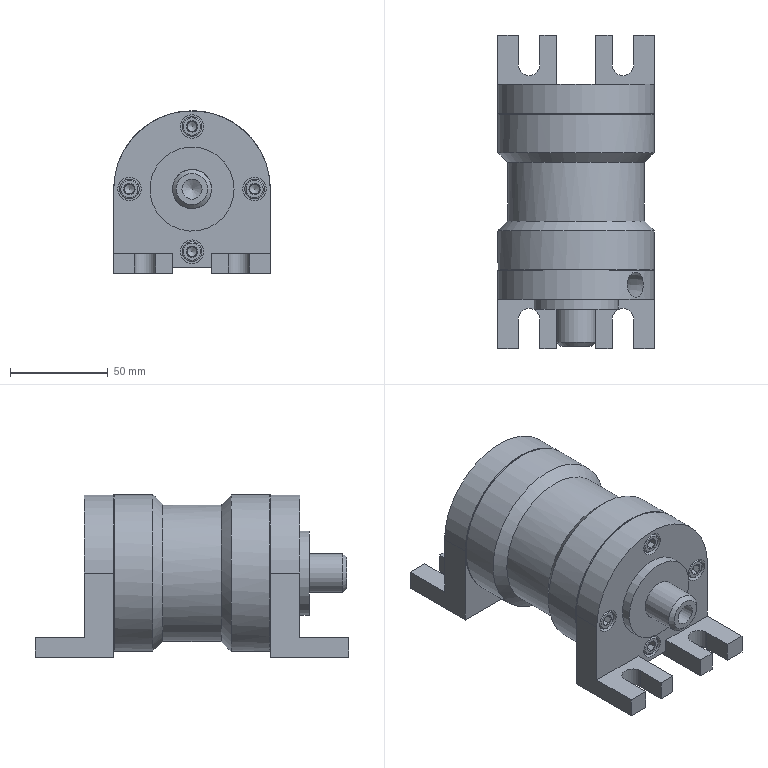Assembly | NX | mm | 29 component files | 29 solids | 459 faces | box 80 x 160 x 83 mm | volume 493574 mm3 | plane 241 | cylinder 109 | cone 90 | torus 19 | commonest cylinder face diameters 6 x16 10 x10 5.795 x8 9.88 x8 6.68 x8 50 x8 7 x8 12 x8
Bill of materials:
unnamed part 1 | 1 |  | L-shaped bracket: an upright plate with a rounded top joined at right angles to a flat foot. The upright has a raised circular boss with a central through hole, and four smaller holes evenly spaced around it. The foot has two open-ended U-slots.
unnamed part 2 | 1 |  | Short cylindrical bushing or pulley-like body with a central through bore and two circumferential grooves on the outside. A smaller-diameter step sits at one end.
unnamed part 3 | 2 |  | Thin torus ring with a round cross-section, consistent with an O-ring shape.
unnamed part 4 | 1 |  | Flat annular disc with a central hole and square edges, consistent with a plain washer.
GB-T97_2-2002,M10 | 1 |  | Thin, flat ring shaped like a plain washer: a circular disc with a concentric round through-hole and a 45-degree-style chamfer around the outer edge on one face.
unnamed part 5 | 2 |  | Very thin flat annular ring with a large central opening and four small holes evenly spaced around it, consistent with a flat gasket or shim.
unnamed part 6 | 1 |  | Hollow cylindrical sleeve with a larger-diameter collar at each end and a reduced-diameter middle section joined by chamfered transitions. One end face has four small holes evenly spaced around it.
unnamed part 7 | 1 |  | Stepped cylindrical shaft or pin. It has a long main diameter with a chamfered end and an axial blind bore at that end, then two progressively smaller steps at the opposite end. The smallest step has a narrow groove.
unnamed part 8 | 1 |  | L-shaped bracket: an upright plate with a rounded top and a flat foot carrying two open U-slots. The upright has a large central hole with hub bosses on both faces, four smaller holes around it, and a transverse hole through the upright's side edge.
GB93-87,6 | 8 |  | Single Coil Spring Lock Washer, Normal Type, GB 93-87,6
unnamed part 9 | 1 |  | Thick disc or nut-like ring with a central through hole and four rectangular notches evenly spaced around the outer rim. Both outer edges are chamfered.
unnamed part 10 | 1 |  | Torus ring with a round cross-section, consistent with an O-ring shape. Its cross-section is thicker relative to its diameter than unnamed part 3.
GB-T70.1-2000,M6x20 | 8 |  | Hexagon Socket Head Cap Screw, GB-T 70.1-2000,M6x20
Mates:
1. fix | Front_cover 1 component
2. touch align | Rear_cover 1 face | Front_cover 1 face
3. distance | Rear_cover 1 face | Front_cover 1 face
4. concentric | Gasket 2 edge | Front_cover 1 edge
5. concentric | Gasket 1 edge | Rear_cover 1 edge
6. concentric | Cylinder_barrel 1 edge | Gasket 2 edge
7. concentric | GB-T97_2-2002_M10 1 edge | Piston 1 edge
8. concentric | Piston_rod 1 edge | Piston 1 edge
9. concentric | Nut_M10 1 edge | GB-T97_2-2002_M10 1 edge
10. touch align | Piston_rod 1 face | Cylinder_barrel 1 face
11. distance | Piston 1 face | Rear_cover 1 face
12. concentric | Washer 1 edge | Piston 1 edge
13. concentric | O_ring 2 edge | Piston 1 edge
14. bond | Piston 1 component | assembly component
15. bond | O_ring 2 component | assembly component
16. bond | O_ring 1 component | assembly component
17. linear | assembly datumaxis | assembly cartesiancoordinatesystem | assembly cartesiancoordinatesystem
18. concentric | GB93-87_6 8 edge | GB-T70_1-2000_M6x20 8 edge
19. concentric | GB93-87_6 8 edge | Front_cover 1 edge
20. concentric | GB-T70_1-2000_M6x20 7 edge | GB93-87_6 7 edge
21. concentric | GB93-87_6 7 edge | Rear_cover 1 edge
22. bond | Cylinder_barrel 1 component | assembly component
23. bond | GB93-87_6 8 component | assembly component
24. bond | GB-T70_1-2000_M6x20 8 component | assembly component
25. bond | GB-T70_1-2000_M6x20 7 component | assembly component
26. bond | GB93-87_6 7 component | assembly component
27. bond | GB93-87_6 6 component | assembly component
28. bond | GB-T70_1-2000_M6x20 6 component | assembly component
29. bond | GB-T70_1-2000_M6x20 5 component | assembly component
30. bond | GB93-87_6 5 component | assembly component
31. bond | GB93-87_6 4 component | assembly component
32. bond | GB-T70_1-2000_M6x20 4 component | assembly component
33. bond | GB-T70_1-2000_M6x20 3 component | assembly component
34. bond | GB93-87_6 3 component | assembly component
35. bond | GB93-87_6 2 component | assembly component
36. bond | GB-T70_1-2000_M6x20 2 component | assembly component
37. bond | GB-T70_1-2000_M6x20 1 component | assembly component
38. bond | GB93-87_6 1 component | assembly component
39. circular | assembly datumaxis | assembly cartesiancoordinatesystem | assembly cartesiancoordinatesystem | assembly cartesiancoordinatesystem | assembly cartesiancoordinatesystem
40. circular | assembly datumaxis | assembly cartesiancoordinatesystem | assembly cartesiancoordinatesystem | assembly cartesiancoordinatesystem | assembly cartesiancoordinatesystem
41. circular | assembly datumaxis | assembly cartesiancoordinatesystem | assembly cartesiancoordinatesystem | assembly cartesiancoordinatesystem | assembly cartesiancoordinatesystem
42. circular | assembly datumaxis | assembly cartesiancoordinatesystem | assembly cartesiancoordinatesystem | assembly cartesiancoordinatesystem | assembly cartesiancoordinatesystem
43. concentric | O_ring_20 1 edge | Front_cover 1 edge